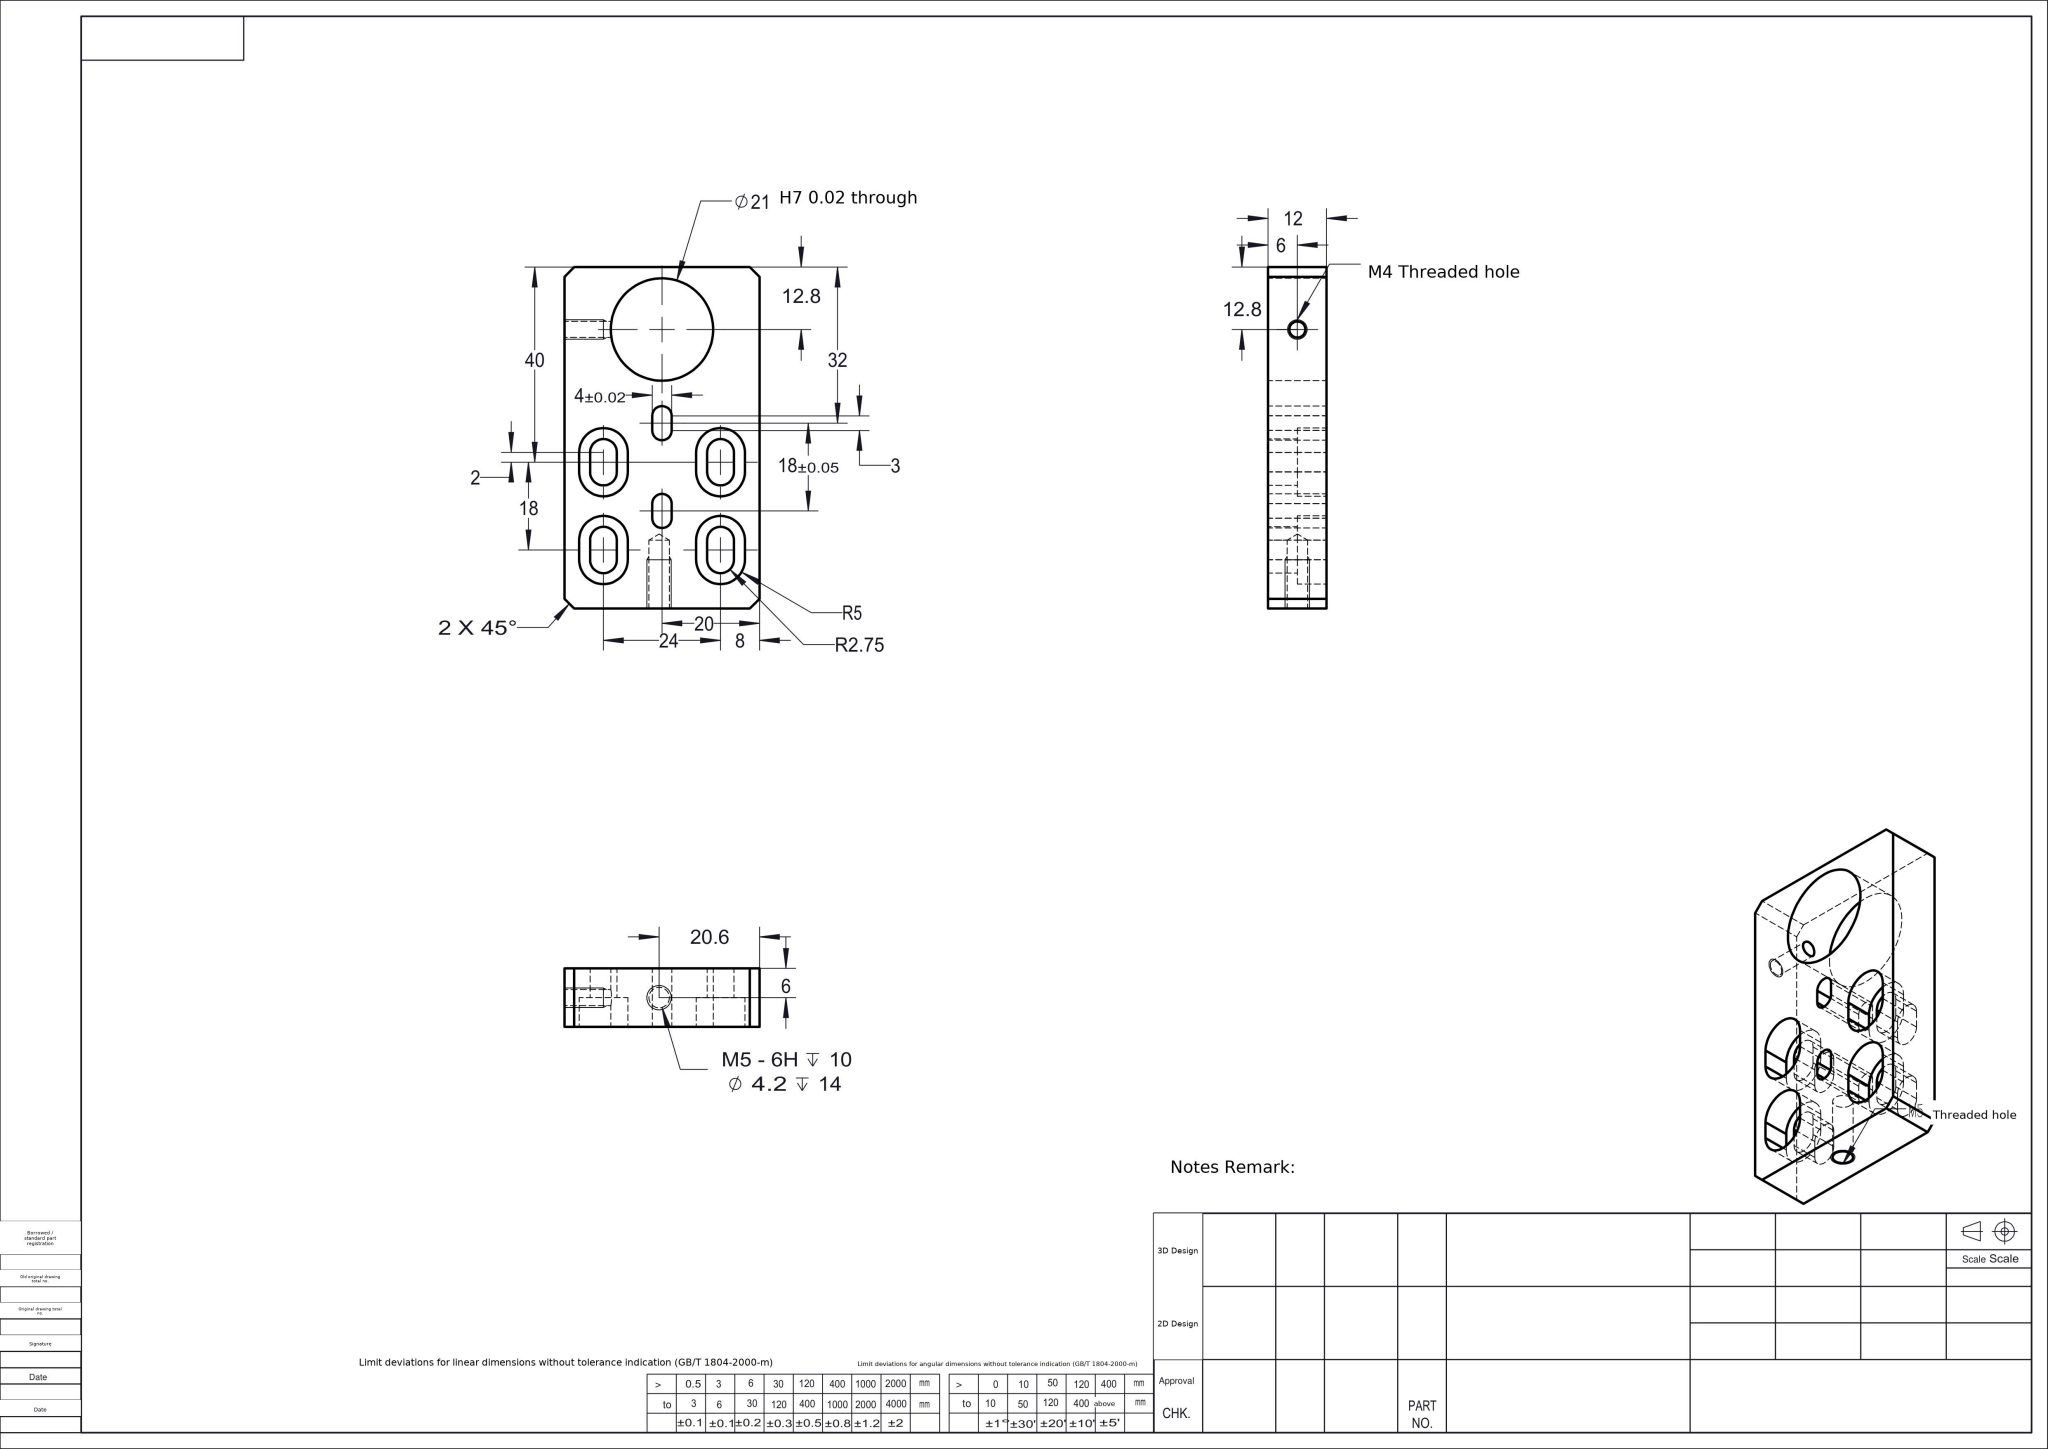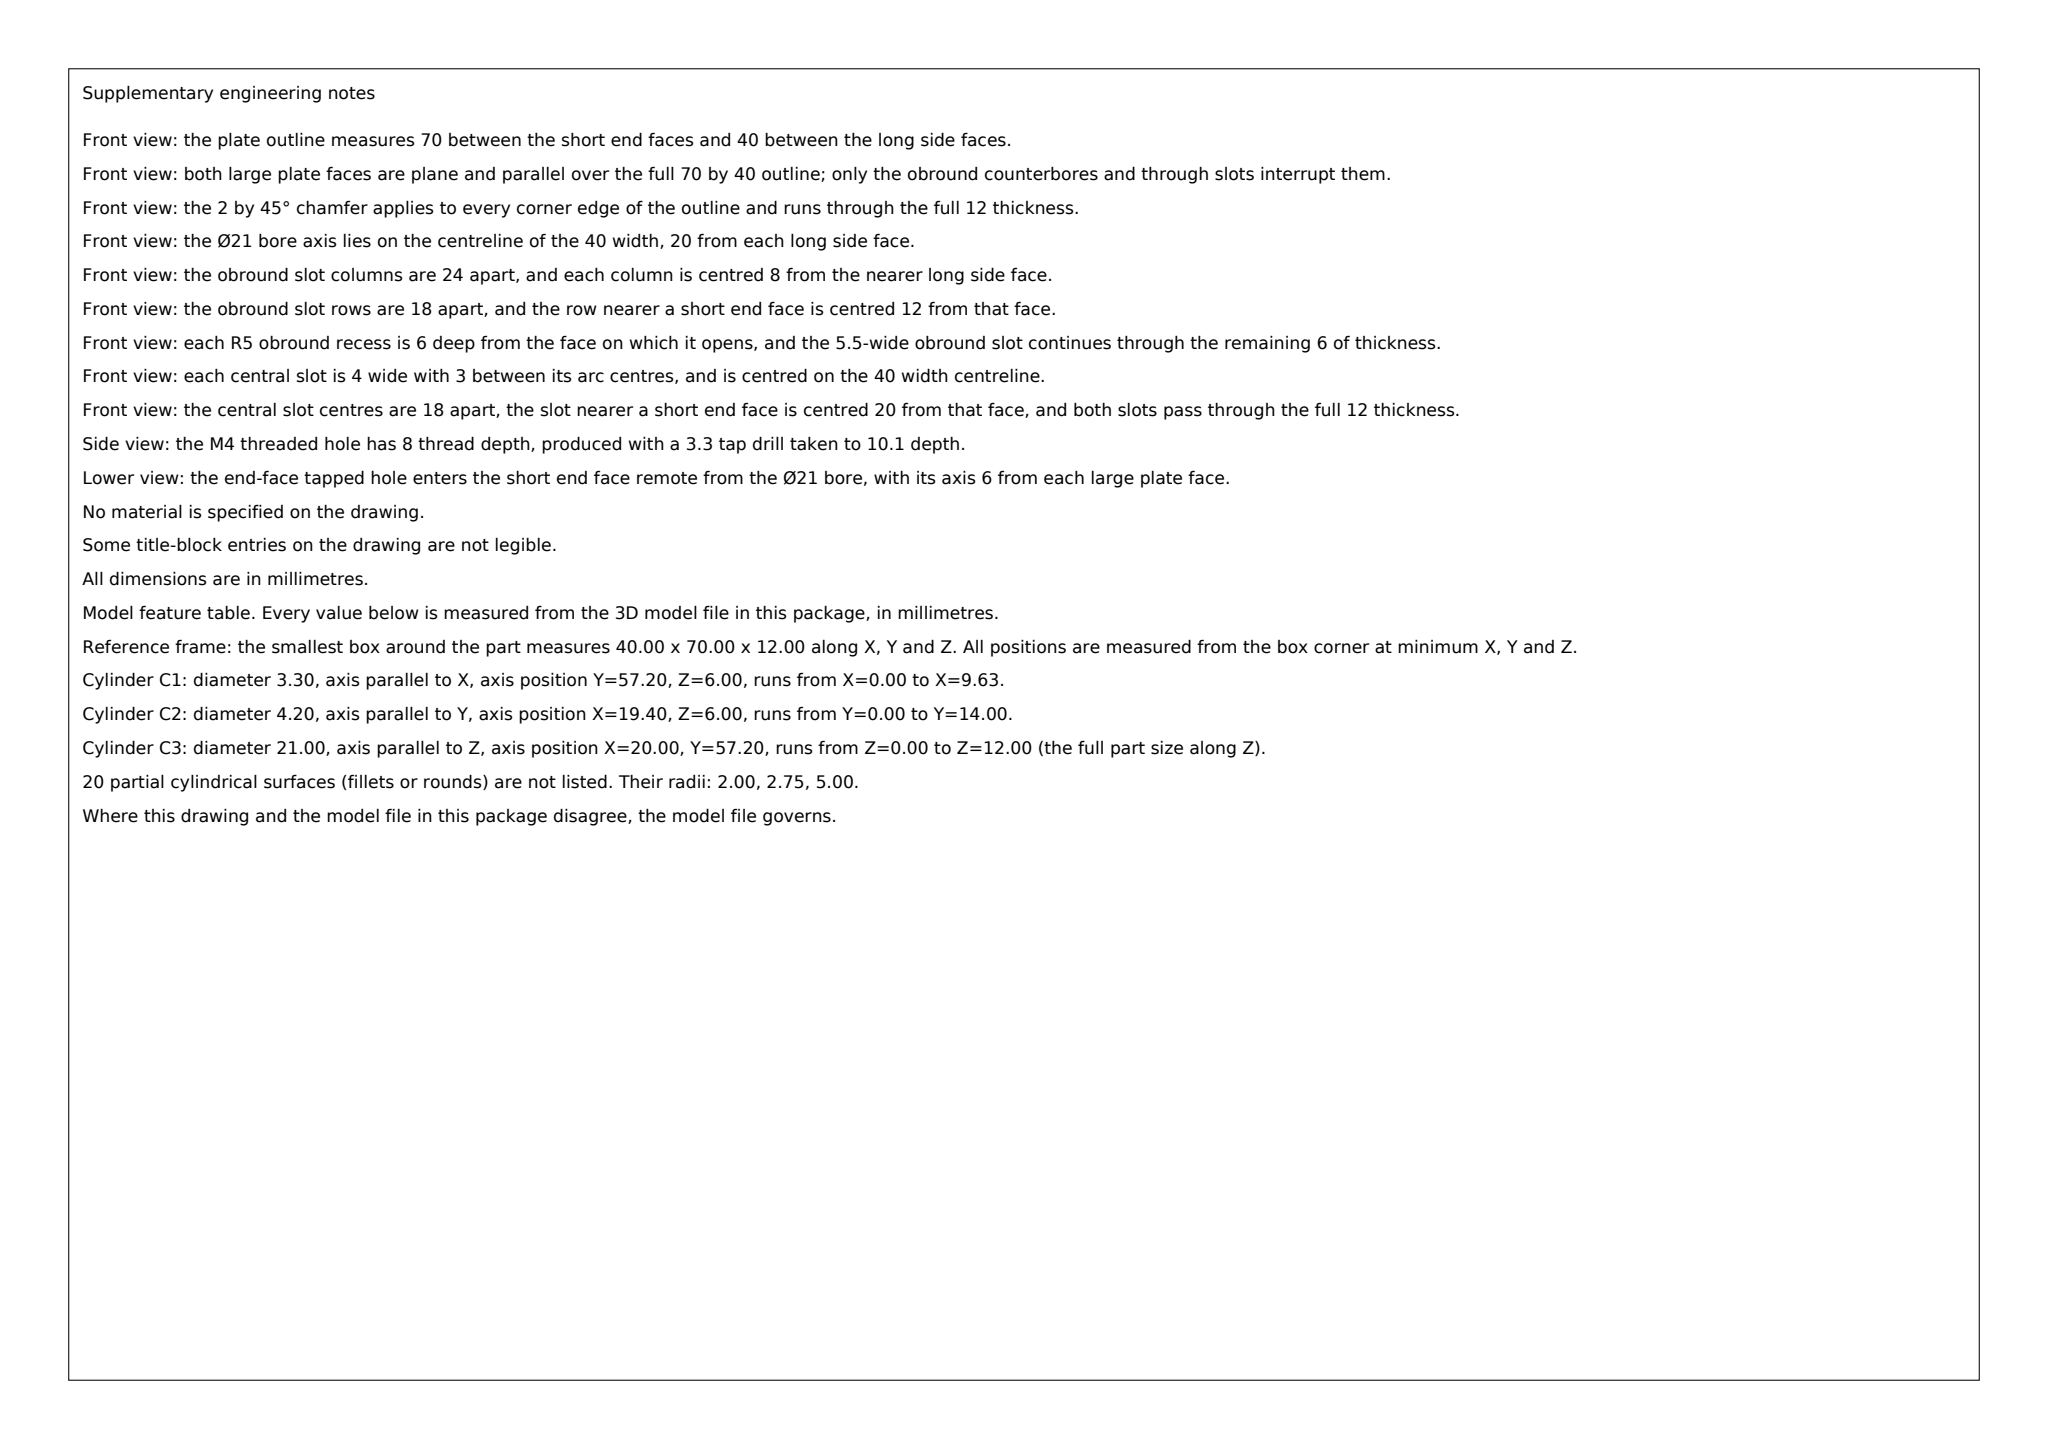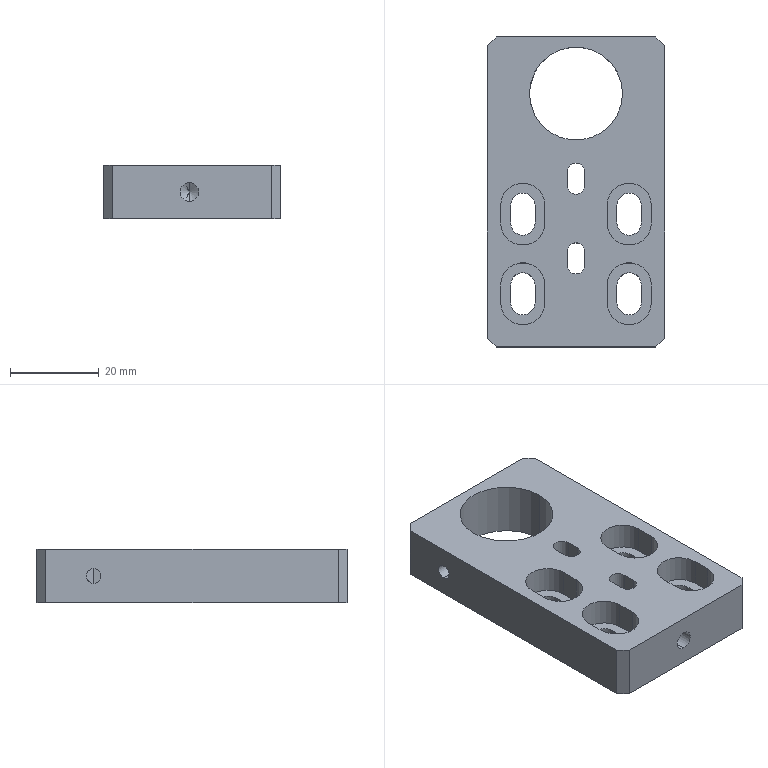Part | SolidWorks | mm | 1 solid | 62 faces | box 40 x 70 x 12 mm | volume 24534 mm3 | plane 34 | cylinder 26 | cone 2 | commonest cylinder face diameters 5.5 x8 10 x8 4 x4 3.3 x2 4.2 x2 21 x2
Drawing notes:
FRONT VIEW: OVERALL HT 70 (TOP EDGE TO BOT EDGE) | from the solid: bbox_xyz Y = 70.0; planes y=0.0 and y=70.0
FRONT VIEW: OVERALL WIDTH 40 (LEFT EDGE TO RIGHT EDGE) | from the solid: bbox_xyz X = 40.0; planes x=0.0 and x=40.0
4X STEPPED SLOT: R5 CBORE DP 6, R2.75 THRU 12 | from the solid: Ø10 cyls len 6 at z0-6 (8/32, 10/14/28/32); Ø5.5 cyls len 6; plate thk 12
M4 THD HOLE: TAP DRILL Ø3.3 DP 9.6, 2X EA SIDE FACE | from the solid: cylinders Ø3.3 axis x, pos y=57.2 z=6.0, length 9.63, count 2
FRONT VIEW: 4X CHAMFER 2 X 45 DEG, ALL FOUR CORNERS | from the solid: Plate bbox 40 x 70 x 12 with no fillet_radii; corner breaks identical at all 4 corners of the 40 x 70 face, matching the single 2 X 45 deg callout
build123d program:
from build123d import *

# Parameters (mm, degrees)
SKETCH1_W             = 40
SKETCH1_H             = 70
BOSS_EXTRUDE1_DEPTH   = 12
CHAMFER1_SIZE         = 2
CUT_EXTRUDE1_DEPTH    = 20
CUT_EXTRUDE2_DEPTH    = 6
CUT_EXTRUDE3_DEPTH    = 20
SKETCH5_R             = 10.5
CUT_EXTRUDE4_DEPTH    = 43.059
M5_TAPPED_HOLE1_D     = 4.2
M5_TAPPED_HOLE1_DEPTH = 14
M5_TAPPED_HOLE1_TIP   = 1.262
M4_TAPPED_HOLE1_D     = 3.3
M4_TAPPED_HOLE1_DEPTH = 10.1
M4_TAPPED_HOLE1_TIP   = 0.9914


with BuildPart() as part:
    # Sketch1 → Boss-Extrude1 (new body)
    with BuildSketch(Plane.XY):
        Rectangle(SKETCH1_W, SKETCH1_H)
    extrude(amount=BOSS_EXTRUDE1_DEPTH)

    # Chamfer1
    chamfer1_edges = [part.edges().sort_by_distance(p)[0] for p in [
        (20, -35, 6),
        (-20, -35, 6),
        (-20, 35, 6),
        (20, 35, 6),
    ]]
    chamfer(chamfer1_edges, length=CHAMFER1_SIZE)

    # Sketch2 → Cut-Extrude1 (cut)
    with BuildSketch(Plane.XY.offset(12)):
        with BuildLine():
            Line((-14.75, -7), (-14.75, -3))
            ThreePointArc((-14.75, -3), (-12, -0.25), (-9.25, -3))
            Line((-9.25, -3), (-9.25, -7))
            ThreePointArc((-9.25, -7), (-12, -9.75), (-14.75, -7))
        make_face()
        with BuildLine():
            Line((14.75, -3), (14.75, -7))
            ThreePointArc((14.75, -7), (12, -9.75), (9.25, -7))
            Line((9.25, -7), (9.25, -3))
            ThreePointArc((9.25, -3), (12, -0.25), (14.75, -3))
        make_face()
        with BuildLine():
            Line((14.75, -21), (14.75, -25))
            ThreePointArc((14.75, -25), (12, -27.75), (9.25, -25))
            Line((9.25, -25), (9.25, -21))
            ThreePointArc((9.25, -21), (12, -18.25), (14.75, -21))
        make_face()
        with BuildLine():
            Line((-9.25, -21), (-9.25, -25))
            ThreePointArc((-9.25, -25), (-12, -27.75), (-14.75, -25))
            Line((-14.75, -25), (-14.75, -21))
            ThreePointArc((-14.75, -21), (-12, -18.25), (-9.25, -21))
        make_face()
    extrude(amount=-CUT_EXTRUDE1_DEPTH, mode=Mode.SUBTRACT)

    # Sketch3 → Cut-Extrude2 (cut)
    with BuildSketch(Plane.XY.offset(12)):
        with BuildLine():
            Line((-7, -3), (-7, -7))
            ThreePointArc((-7, -7), (-12, -12), (-17, -7))
            Line((-17, -7), (-17, -3))
            ThreePointArc((-17, -3), (-12, 2), (-7, -3))
        make_face()
        with BuildLine():
            Line((17, -3), (17, -7))
            ThreePointArc((17, -7), (12, -12), (7, -7))
            Line((7, -7), (7, -3))
            ThreePointArc((7, -3), (12, 2), (17, -3))
        make_face()
        with BuildLine():
            Line((17, -21), (17, -25))
            ThreePointArc((17, -25), (12, -30), (7, -25))
            Line((7, -25), (7, -21))
            ThreePointArc((7, -21), (12, -16), (17, -21))
        make_face()
        with BuildLine():
            Line((-7, -21), (-7, -25))
            ThreePointArc((-7, -25), (-12, -30), (-17, -25))
            Line((-17, -25), (-17, -21))
            ThreePointArc((-17, -21), (-12, -16), (-7, -21))
        make_face()
    extrude(amount=-CUT_EXTRUDE2_DEPTH, mode=Mode.SUBTRACT)

    # Sketch4 → Cut-Extrude3 (cut)
    with BuildSketch(Plane.XY.offset(12)):
        with BuildLine():
            Line((2, 4.5), (2, 1.5))
            ThreePointArc((2, 1.5), (0, -0.5), (-2, 1.5))
            Line((-2, 1.5), (-2, 4.5))
            ThreePointArc((-2, 4.5), (0, 6.5), (2, 4.5))
        make_face()
        with BuildLine():
            Line((2, -13.5), (2, -16.5))
            ThreePointArc((2, -16.5), (0, -18.5), (-2, -16.5))
            Line((-2, -16.5), (-2, -13.5))
            ThreePointArc((-2, -13.5), (0, -11.5), (2, -13.5))
        make_face()
    extrude(amount=-CUT_EXTRUDE3_DEPTH, mode=Mode.SUBTRACT)

    # Sketch5 → Cut-Extrude4 (cut, through all)
    with BuildSketch(Plane(origin=(0, 0, 0), x_dir=(-1, 0, 0), z_dir=(0, 0, -1))):
        with Locations((0, 22.202)):
            Circle(SKETCH5_R)
    extrude(amount=-CUT_EXTRUDE4_DEPTH, mode=Mode.SUBTRACT)

    # M5 Tapped Hole1
    with Locations(Plane(origin=(0, -35, 0), x_dir=(-1, 0, 0), z_dir=(0, -1, 0))):
        with Locations((0.6, -6)):
            Hole(M5_TAPPED_HOLE1_D / 2, depth=M5_TAPPED_HOLE1_DEPTH)
            with Locations((0, 0, -(M5_TAPPED_HOLE1_DEPTH + M5_TAPPED_HOLE1_TIP / 2))):  # 118° drill point
                Cone(0, M5_TAPPED_HOLE1_D / 2, M5_TAPPED_HOLE1_TIP, mode=Mode.SUBTRACT)

    # M4 Tapped Hole1
    with Locations(Plane.ZY.offset(20)):
        with Locations((6, 22.202)):
            Hole(M4_TAPPED_HOLE1_D / 2, depth=M4_TAPPED_HOLE1_DEPTH)
            with Locations((0, 0, -(M4_TAPPED_HOLE1_DEPTH + M4_TAPPED_HOLE1_TIP / 2))):  # 118° drill point
                Cone(0, M4_TAPPED_HOLE1_D / 2, M4_TAPPED_HOLE1_TIP, mode=Mode.SUBTRACT)


solid = part.part